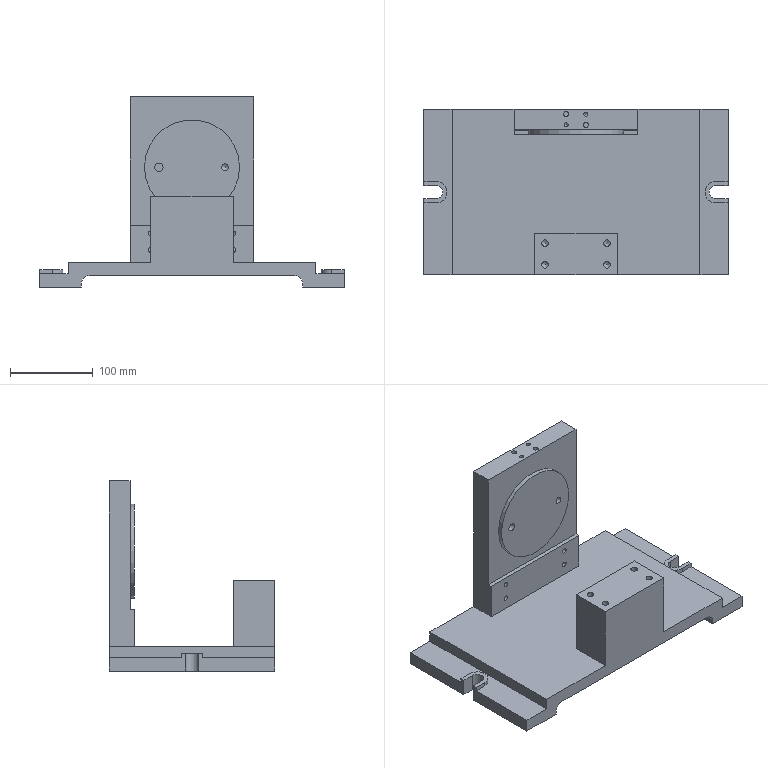Component | NX | FIXTURE_BODY | 1 solid | 72 faces | volume 2496909 mm3 | plane 42 | cylinder 21 | cone 9 | commonest cylinder face diameters 6 x6 8 x5 5 x2 16 x2 26 x2 20 x2 115 x1 10 x1